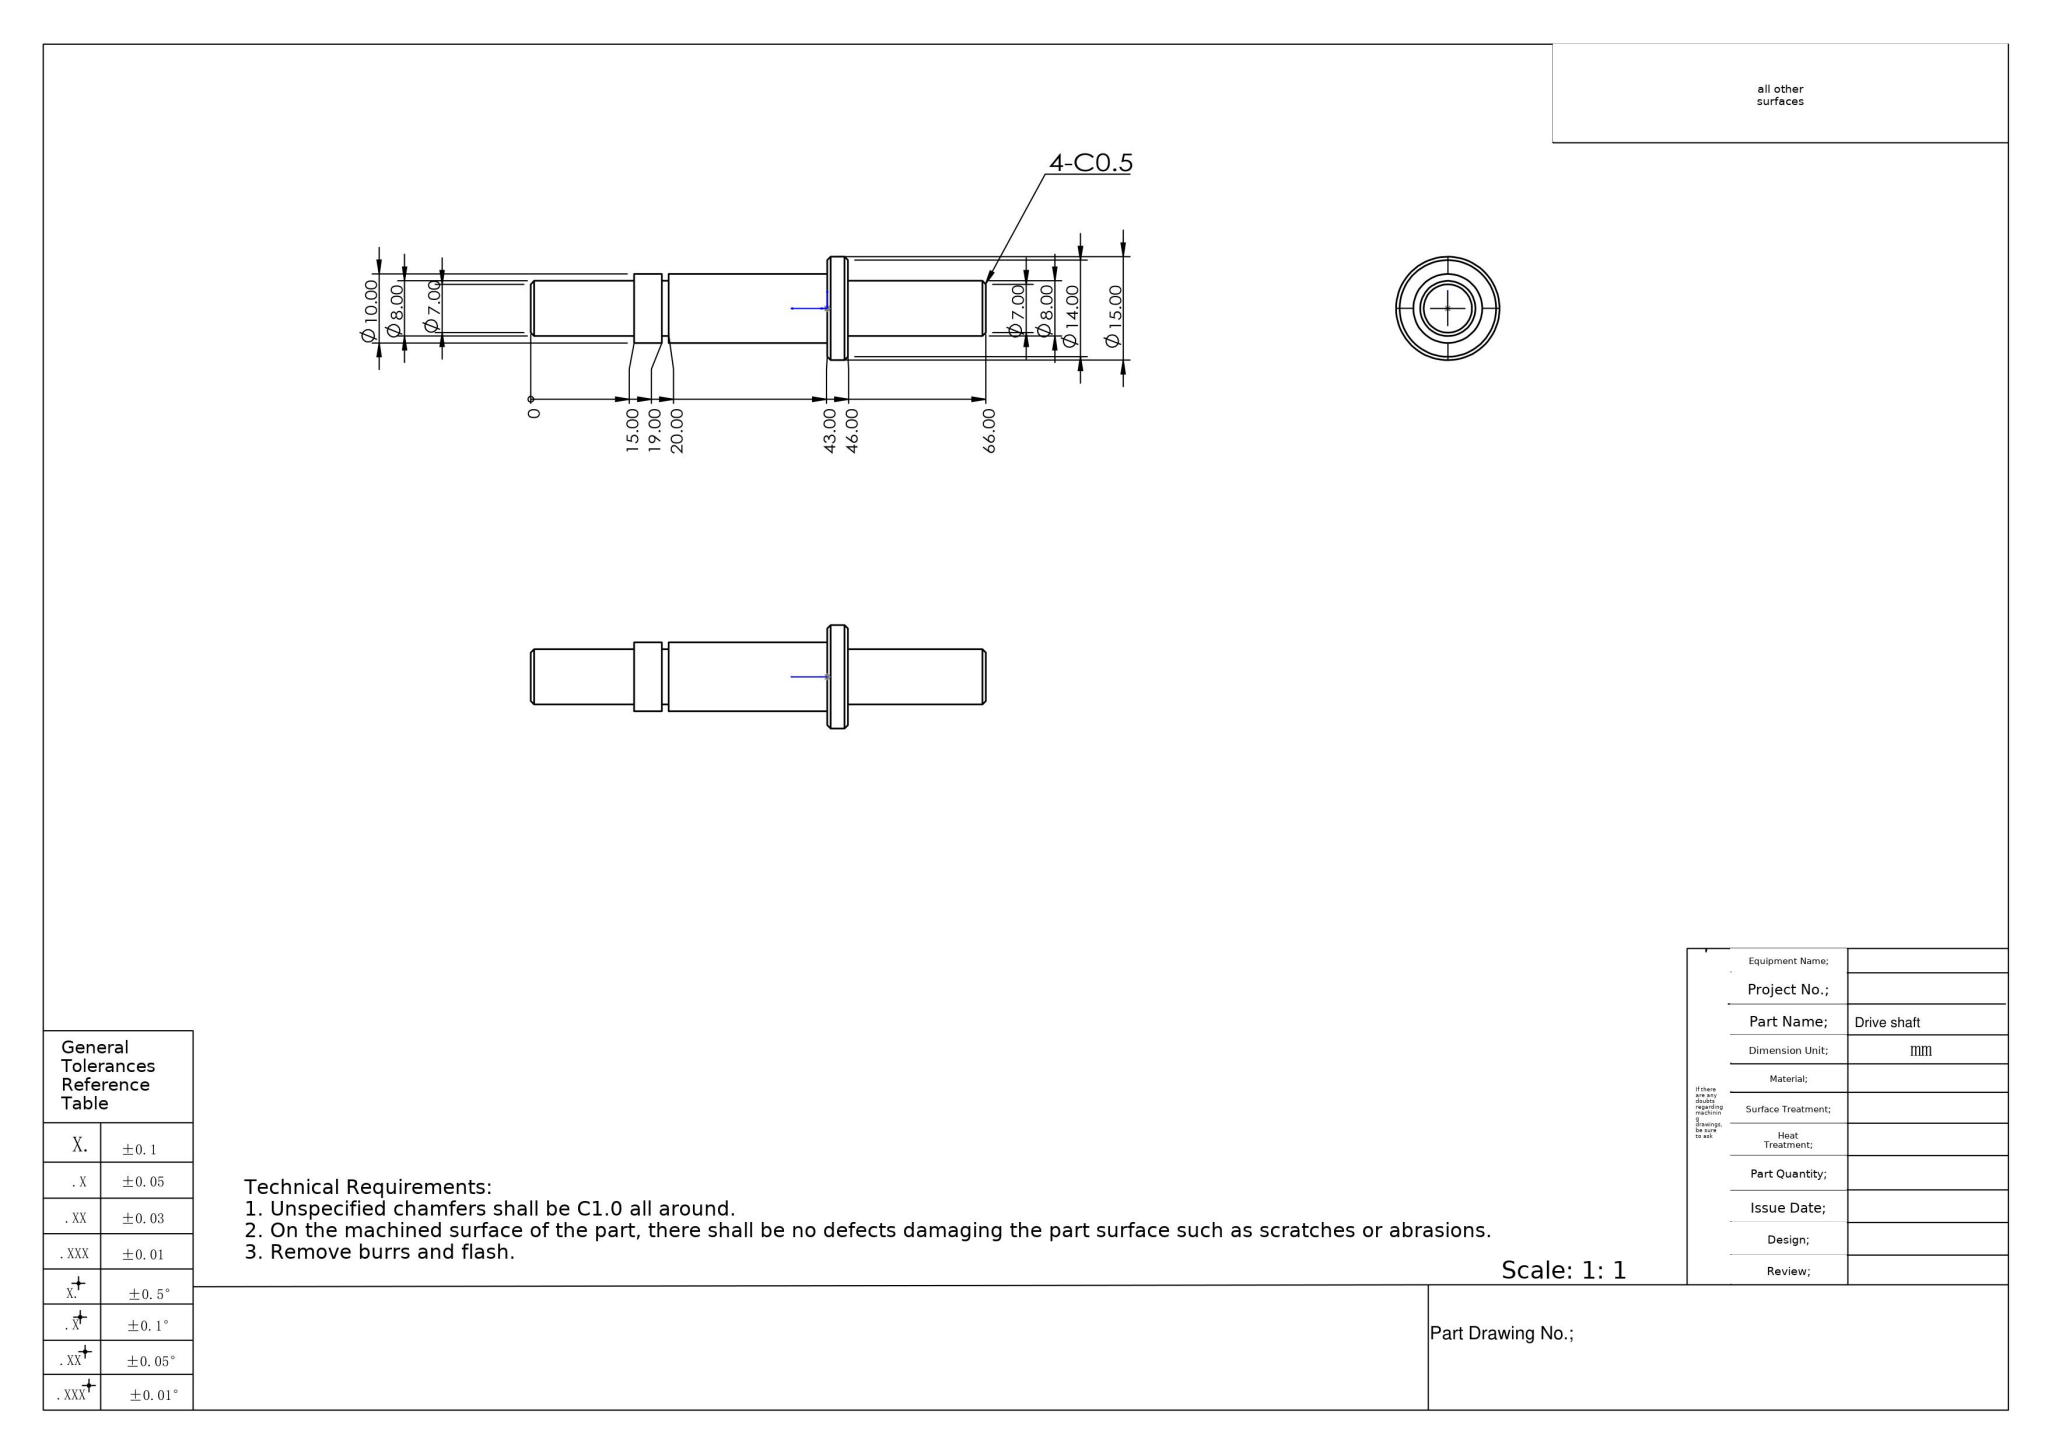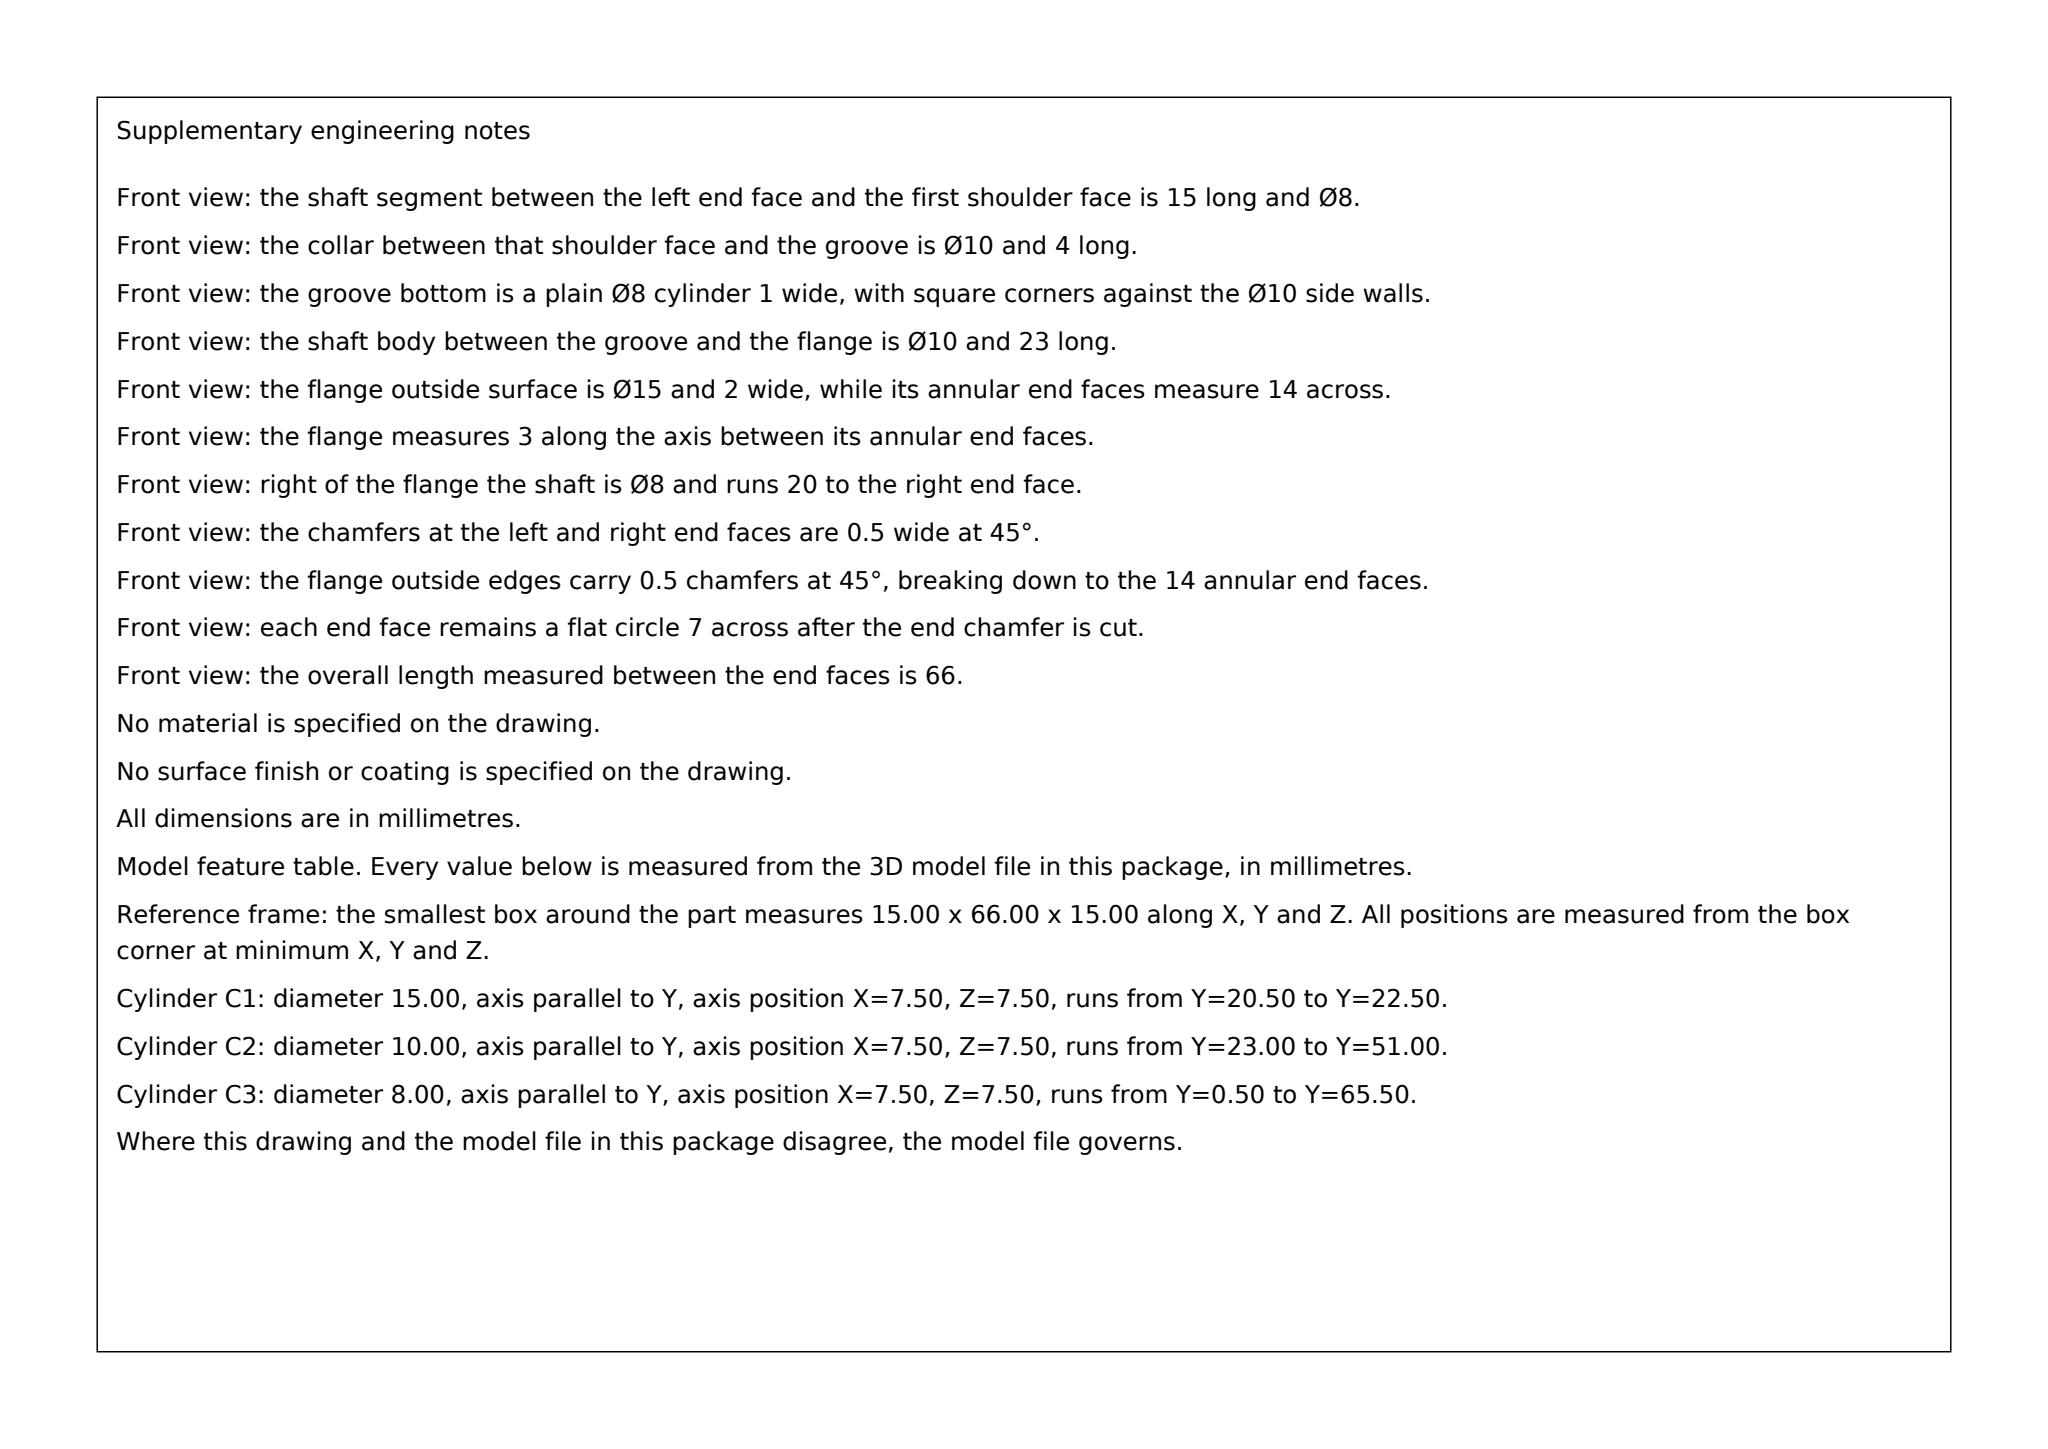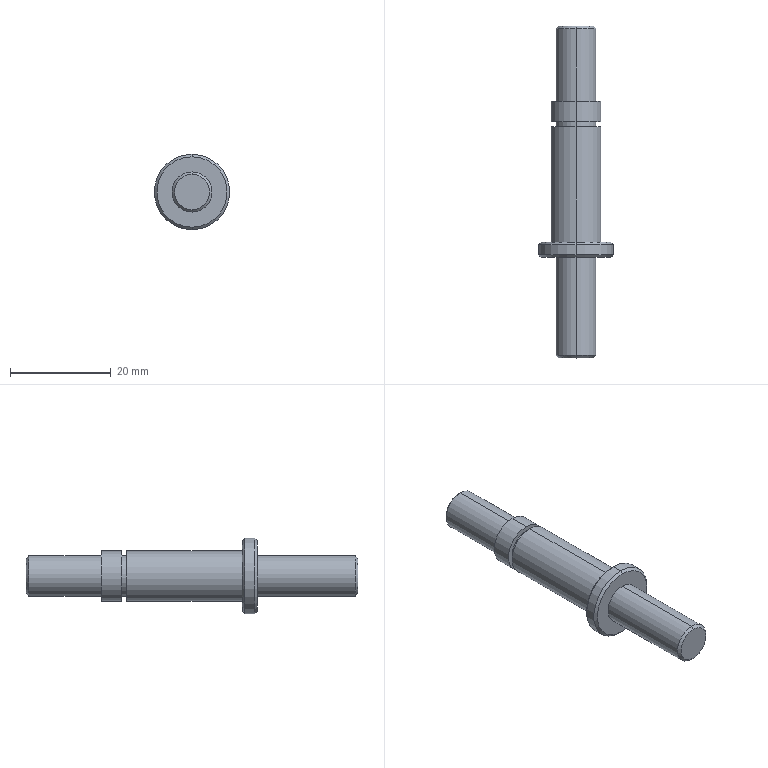Part | SolidWorks | mm | 1 solid | 27 faces | box 15 x 66 x 15 mm | volume 4443 mm3 | cylinder 12 | cone 8 | plane 7 | commonest cylinder face diameters 8 x6 10 x4 15 x2
build123d program:
from build123d import *

# Parameters (mm, degrees)
SKETCH1_R           = 5
BOSS_EXTRUDE1_DEPTH = 28
SKETCH2_R           = 7.5
BOSS_EXTRUDE2_DEPTH = 3
CHAMFER1_SIZE       = 0.5
SKETCH3_R           = 4
BOSS_EXTRUDE3_DEPTH = 20
CHAMFER2_SIZE       = 0.5
BOSS_EXTRUDE4_START = 15
SKETCH4_R           = 4
BOSS_EXTRUDE4_DEPTH = 15
CHAMFER3_SIZE       = 0.5
SKETCH5_W           = 1
SKETCH5_H           = 1


with BuildPart() as part:
    # Sketch1 → Boss-Extrude1 (new body)
    with BuildSketch(Plane(origin=(0, 0, 0), x_dir=(1, 0, 0), z_dir=(0, 1, 0))):
        with Locations(Location((0, 0, 0), (0, 0, 270))):
            Circle(SKETCH1_R)
    extrude(amount=BOSS_EXTRUDE1_DEPTH)

    # Sketch2 → Boss-Extrude2 (add)
    with BuildSketch(Plane.XZ):
        with Locations(Location((0, 0, 0), (0, 0, 270))):
            Circle(SKETCH2_R)
    extrude(amount=BOSS_EXTRUDE2_DEPTH)

    # Chamfer1
    chamfer1_edges = [part.edges().sort_by_distance(p)[0] for p in [
        (0, 0, 7.5),
        (0, -3, 7.5),
    ]]
    chamfer(chamfer1_edges, length=CHAMFER1_SIZE)

    # Sketch3 → Boss-Extrude3 (add)
    with BuildSketch(Plane.XZ.offset(3)):
        with Locations(Location((0, 0, 0), (0, 0, 270))):
            Circle(SKETCH3_R)
    extrude(amount=BOSS_EXTRUDE3_DEPTH)

    # Chamfer2
    chamfer2_edges = [part.edges().sort_by_distance(p)[0] for p in [
        (0, -23, 4),
    ]]
    chamfer(chamfer2_edges, length=CHAMFER2_SIZE)

    # Sketch4 → Boss-Extrude4 (add)
    with BuildSketch(Plane(origin=(0, 28, 0), x_dir=(1, 0, 0), z_dir=(0, 1, 0)).offset(BOSS_EXTRUDE4_START)):
        with Locations(Location((0, 0, 0), (0, 0, 90))):
            Circle(SKETCH4_R)
    extrude(amount=-BOSS_EXTRUDE4_DEPTH)

    # Chamfer3
    chamfer3_edges = [part.edges().sort_by_distance(p)[0] for p in [
        (0, 43, 4),
    ]]
    chamfer(chamfer3_edges, length=CHAMFER3_SIZE)

    # Sketch5 → Cut-Revolve1 (revolve, cut)
    with BuildSketch(Plane(origin=(0, 0, 0), x_dir=(0, 0, -1), z_dir=(1, 0, 0)), mode=Mode.PRIVATE) as cut_revolve1_sk:
        with Locations((-4.5, 23.5)):
            Rectangle(SKETCH5_W, SKETCH5_H)
    revolve(cut_revolve1_sk.sketch.rotate(Axis((0, 0, 0), (0, 1, 0)), 180), axis=Axis((0, 0, 0), (0, 1, 0)), mode=Mode.SUBTRACT)


solid = part.part
STEP:
#1=CARTESIAN_POINT('',(0.,28.,5.));
#2=VERTEX_POINT('',#1);
#3=CARTESIAN_POINT('',(0.,28.,-5.));
#4=VERTEX_POINT('',#3);
#5=CARTESIAN_POINT('',(0.,28.,0.));
#6=DIRECTION('',(0.,1.,0.));
#7=DIRECTION('',(0.,0.,1.));
#8=AXIS2_PLACEMENT_3D('',#5,#6,#7);
#9=CIRCLE('',#8,5.);
#10=EDGE_CURVE('',#2,#4,#9,.T.);
#11=ORIENTED_EDGE('',*,*,#10,.F.);
#12=CARTESIAN_POINT('',(0.,24.,5.));
#13=VERTEX_POINT('',#12);
#14=CARTESIAN_POINT('',(0.,28.,5.));
#15=DIRECTION('',(0.,-1.,0.));
#16=VECTOR('',#15,1000.);
#17=LINE('',#14,#16);
#18=EDGE_CURVE('',#2,#13,#17,.T.);
#19=ORIENTED_EDGE('',*,*,#18,.T.);
#20=CARTESIAN_POINT('',(0.,24.,-5.));
#21=VERTEX_POINT('',#20);
#22=CARTESIAN_POINT('',(0.,24.,0.));
#23=DIRECTION('',(0.,-1.,0.));
#24=DIRECTION('',(0.,0.,-1.));
#25=AXIS2_PLACEMENT_3D('',#22,#23,#24);
#26=CIRCLE('',#25,5.);
#27=EDGE_CURVE('',#21,#13,#26,.T.);
#28=ORIENTED_EDGE('',*,*,#27,.F.);
#29=CARTESIAN_POINT('',(0.,28.,-5.));
#30=DIRECTION('',(0.,-1.,0.));
#31=VECTOR('',#30,1000.);
#32=LINE('',#29,#31);
#33=EDGE_CURVE('',#4,#21,#32,.T.);
#34=ORIENTED_EDGE('',*,*,#33,.F.);
#35=EDGE_LOOP('',(#11,#19,#28,#34));
#36=FACE_OUTER_BOUND('',#35,.T.);
#37=CARTESIAN_POINT('',(0.,28.,0.));
#38=DIRECTION('',(0.,-1.,0.));
#39=DIRECTION('',(0.,0.,-1.));
#40=AXIS2_PLACEMENT_3D('',#37,#38,#39);
#41=CYLINDRICAL_SURFACE('',#40,5.);
#42=ADVANCED_FACE('',(#36),#41,.T.);
#43=CARTESIAN_POINT('',(0.,42.5,-4.));
#44=VERTEX_POINT('',#43);
#45=CARTESIAN_POINT('',(0.,42.5,4.));
#46=VERTEX_POINT('',#45);
#47=CARTESIAN_POINT('',(0.,42.5,0.));
#48=DIRECTION('',(0.,-1.,0.));
#49=DIRECTION('',(0.,0.,1.));
#50=AXIS2_PLACEMENT_3D('',#47,#48,#49);
#51=CIRCLE('',#50,4.);
#52=EDGE_CURVE('',#44,#46,#51,.T.);
#53=ORIENTED_EDGE('',*,*,#52,.T.);
#54=CARTESIAN_POINT('',(0.,28.,4.));
#55=VERTEX_POINT('',#54);
#56=CARTESIAN_POINT('',(0.,43.,4.));
#57=DIRECTION('',(0.,-1.,0.));
#58=VECTOR('',#57,1000.);
#59=LINE('',#56,#58);
#60=EDGE_CURVE('',#46,#55,#59,.T.);
#61=ORIENTED_EDGE('',*,*,#60,.T.);
#62=CARTESIAN_POINT('',(0.,28.,-4.));
#63=VERTEX_POINT('',#62);
#64=CARTESIAN_POINT('',(0.,28.,0.));
#65=DIRECTION('',(0.,1.,0.));
#66=DIRECTION('',(0.,0.,1.));
#67=AXIS2_PLACEMENT_3D('',#64,#65,#66);
#68=CIRCLE('',#67,4.);
#69=EDGE_CURVE('',#55,#63,#68,.T.);
#70=ORIENTED_EDGE('',*,*,#69,.T.);
#71=CARTESIAN_POINT('',(0.,43.,-4.));
#72=DIRECTION('',(0.,-1.,0.));
#73=VECTOR('',#72,1000.);
#74=LINE('',#71,#73);
#75=EDGE_CURVE('',#44,#63,#74,.T.);
#76=ORIENTED_EDGE('',*,*,#75,.F.);
#77=EDGE_LOOP('',(#53,#61,#70,#76));
#78=FACE_OUTER_BOUND('',#77,.T.);
#79=CARTESIAN_POINT('',(0.,43.,0.));
#80=DIRECTION('',(0.,-1.,0.));
#81=DIRECTION('',(0.,0.,-1.));
#82=AXIS2_PLACEMENT_3D('',#79,#80,#81);
#83=CYLINDRICAL_SURFACE('',#82,4.);
#84=ADVANCED_FACE('',(#78),#83,.T.);
#85=CARTESIAN_POINT('',(0.,43.,3.5));
#86=VERTEX_POINT('',#85);
#87=CARTESIAN_POINT('',(0.,43.,-3.5));
#88=VERTEX_POINT('',#87);
#89=CARTESIAN_POINT('',(0.,43.,0.));
#90=DIRECTION('',(0.,1.,0.));
#91=DIRECTION('',(0.,0.,1.));
#92=AXIS2_PLACEMENT_3D('',#89,#90,#91);
#93=CIRCLE('',#92,3.5);
#94=EDGE_CURVE('',#86,#88,#93,.T.);
#95=ORIENTED_EDGE('',*,*,#94,.F.);
#96=CARTESIAN_POINT('',(0.,43.,3.5));
#97=DIRECTION('',(0.,-0.7071,0.7071));
#98=VECTOR('',#97,1000.);
#99=LINE('',#96,#98);
#100=EDGE_CURVE('',#86,#46,#99,.T.);
#101=ORIENTED_EDGE('',*,*,#100,.T.);
#102=ORIENTED_EDGE('',*,*,#52,.F.);
#103=CARTESIAN_POINT('',(0.,43.,-3.5));
#104=DIRECTION('',(0.,-0.7071,-0.7071));
#105=VECTOR('',#104,1000.);
#106=LINE('',#103,#105);
#107=EDGE_CURVE('',#88,#44,#106,.T.);
#108=ORIENTED_EDGE('',*,*,#107,.F.);
#109=EDGE_LOOP('',(#95,#101,#102,#108));
#110=FACE_OUTER_BOUND('',#109,.T.);
#111=CARTESIAN_POINT('',(0.,43.,0.));
#112=DIRECTION('',(0.,-1.,0.));
#113=DIRECTION('',(0.,0.,-1.));
#114=AXIS2_PLACEMENT_3D('',#111,#112,#113);
#115=CONICAL_SURFACE('',#114,3.5,0.7854);
#116=ADVANCED_FACE('',(#110),#115,.T.);
#117=CARTESIAN_POINT('',(0.,24.,-4.));
#118=VERTEX_POINT('',#117);
#119=CARTESIAN_POINT('',(0.,24.,4.));
#120=VERTEX_POINT('',#119);
#121=CARTESIAN_POINT('',(0.,24.,0.));
#122=DIRECTION('',(0.,-1.,0.));
#123=DIRECTION('',(0.,0.,-1.));
#124=AXIS2_PLACEMENT_3D('',#121,#122,#123);
#125=CIRCLE('',#124,4.);
#126=EDGE_CURVE('',#118,#120,#125,.T.);
#127=ORIENTED_EDGE('',*,*,#126,.T.);
#128=CARTESIAN_POINT('',(0.,23.,4.));
#129=VERTEX_POINT('',#128);
#130=CARTESIAN_POINT('',(0.,0.,4.));
#131=DIRECTION('',(0.,-1.,0.));
#132=VECTOR('',#131,1000.);
#133=LINE('',#130,#132);
#134=EDGE_CURVE('',#120,#129,#133,.T.);
#135=ORIENTED_EDGE('',*,*,#134,.T.);
#136=CARTESIAN_POINT('',(0.,23.,-4.));
#137=VERTEX_POINT('',#136);
#138=CARTESIAN_POINT('',(0.,23.,0.));
#139=DIRECTION('',(0.,-1.,0.));
#140=DIRECTION('',(0.,0.,-1.));
#141=AXIS2_PLACEMENT_3D('',#138,#139,#140);
#142=CIRCLE('',#141,4.);
#143=EDGE_CURVE('',#137,#129,#142,.T.);
#144=ORIENTED_EDGE('',*,*,#143,.F.);
#145=CARTESIAN_POINT('',(0.,0.,-4.));
#146=DIRECTION('',(0.,-1.,0.));
#147=VECTOR('',#146,1000.);
#148=LINE('',#145,#147);
#149=EDGE_CURVE('',#118,#137,#148,.T.);
#150=ORIENTED_EDGE('',*,*,#149,.F.);
#151=EDGE_LOOP('',(#127,#135,#144,#150));
#152=FACE_OUTER_BOUND('',#151,.T.);
#153=CARTESIAN_POINT('',(0.,0.,0.));
#154=DIRECTION('',(0.,-1.,0.));
#155=DIRECTION('',(0.,0.,-1.));
#156=AXIS2_PLACEMENT_3D('',#153,#154,#155);
#157=CYLINDRICAL_SURFACE('',#156,4.);
#158=ADVANCED_FACE('',(#152),#157,.T.);
#159=CARTESIAN_POINT('',(0.,-23.,-3.5));
#160=VERTEX_POINT('',#159);
#161=CARTESIAN_POINT('',(0.,-23.,3.5));
#162=VERTEX_POINT('',#161);
#163=CARTESIAN_POINT('',(0.,-23.,0.));
#164=DIRECTION('',(0.,-1.,0.));
#165=DIRECTION('',(0.,0.,-1.));
#166=AXIS2_PLACEMENT_3D('',#163,#164,#165);
#167=CIRCLE('',#166,3.5);
#168=EDGE_CURVE('',#160,#162,#167,.T.);
#169=ORIENTED_EDGE('',*,*,#168,.F.);
#170=CARTESIAN_POINT('',(0.,-22.5,-4.));
#171=VERTEX_POINT('',#170);
#172=CARTESIAN_POINT('',(0.,-23.,-3.5));
#173=DIRECTION('',(0.,0.7071,-0.7071));
#174=VECTOR('',#173,1000.);
#175=LINE('',#172,#174);
#176=EDGE_CURVE('',#160,#171,#175,.T.);
#177=ORIENTED_EDGE('',*,*,#176,.T.);
#178=CARTESIAN_POINT('',(0.,-22.5,4.));
#179=VERTEX_POINT('',#178);
#180=CARTESIAN_POINT('',(0.,-22.5,0.));
#181=DIRECTION('',(0.,1.,0.));
#182=DIRECTION('',(0.,0.,-1.));
#183=AXIS2_PLACEMENT_3D('',#180,#181,#182);
#184=CIRCLE('',#183,4.);
#185=EDGE_CURVE('',#179,#171,#184,.T.);
#186=ORIENTED_EDGE('',*,*,#185,.F.);
#187=CARTESIAN_POINT('',(0.,-23.,3.5));
#188=DIRECTION('',(0.,0.7071,0.7071));
#189=VECTOR('',#188,1000.);
#190=LINE('',#187,#189);
#191=EDGE_CURVE('',#162,#179,#190,.T.);
#192=ORIENTED_EDGE('',*,*,#191,.F.);
#193=EDGE_LOOP('',(#169,#177,#186,#192));
#194=FACE_OUTER_BOUND('',#193,.T.);
#195=CARTESIAN_POINT('',(0.,-23.,0.));
#196=DIRECTION('',(0.,1.,0.));
#197=DIRECTION('',(0.,0.,1.));
#198=AXIS2_PLACEMENT_3D('',#195,#196,#197);
#199=CONICAL_SURFACE('',#198,3.5,0.7854);
#200=ADVANCED_FACE('',(#194),#199,.T.);
#201=ORIENTED_EDGE('',*,*,#185,.T.);
#202=CARTESIAN_POINT('',(0.,-3.,-4.));
#203=VERTEX_POINT('',#202);
#204=CARTESIAN_POINT('',(0.,-23.,-4.));
#205=DIRECTION('',(0.,1.,0.));
#206=VECTOR('',#205,1000.);
#207=LINE('',#204,#206);
#208=EDGE_CURVE('',#171,#203,#207,.T.);
#209=ORIENTED_EDGE('',*,*,#208,.T.);
#210=CARTESIAN_POINT('',(0.,-3.,4.));
#211=VERTEX_POINT('',#210);
#212=CARTESIAN_POINT('',(0.,-3.,0.));
#213=DIRECTION('',(0.,-1.,0.));
#214=DIRECTION('',(0.,0.,-1.));
#215=AXIS2_PLACEMENT_3D('',#212,#213,#214);
#216=CIRCLE('',#215,4.);
#217=EDGE_CURVE('',#203,#211,#216,.T.);
#218=ORIENTED_EDGE('',*,*,#217,.T.);
#219=CARTESIAN_POINT('',(0.,-23.,4.));
#220=DIRECTION('',(0.,1.,0.));
#221=VECTOR('',#220,1000.);
#222=LINE('',#219,#221);
#223=EDGE_CURVE('',#179,#211,#222,.T.);
#224=ORIENTED_EDGE('',*,*,#223,.F.);
#225=EDGE_LOOP('',(#201,#209,#218,#224));
#226=FACE_OUTER_BOUND('',#225,.T.);
#227=CARTESIAN_POINT('',(0.,-23.,0.));
#228=DIRECTION('',(0.,1.,0.));
#229=DIRECTION('',(0.,0.,1.));
#230=AXIS2_PLACEMENT_3D('',#227,#228,#229);
#231=CYLINDRICAL_SURFACE('',#230,4.);
#232=ADVANCED_FACE('',(#226),#231,.T.);
#233=CARTESIAN_POINT('',(0.,-3.,-7.));
#234=VERTEX_POINT('',#233);
#235=CARTESIAN_POINT('',(0.,-3.,7.));
#236=VERTEX_POINT('',#235);
#237=CARTESIAN_POINT('',(0.,-3.,0.));
#238=DIRECTION('',(0.,-1.,0.));
#239=DIRECTION('',(0.,0.,-1.));
#240=AXIS2_PLACEMENT_3D('',#237,#238,#239);
#241=CIRCLE('',#240,7.);
#242=EDGE_CURVE('',#234,#236,#241,.T.);
#243=ORIENTED_EDGE('',*,*,#242,.F.);
#244=CARTESIAN_POINT('',(0.,-2.5,-7.5));
#245=VERTEX_POINT('',#244);
#246=CARTESIAN_POINT('',(0.,-3.,-7.));
#247=DIRECTION('',(0.,0.7071,-0.7071));
#248=VECTOR('',#247,1000.);
#249=LINE('',#246,#248);
#250=EDGE_CURVE('',#234,#245,#249,.T.);
#251=ORIENTED_EDGE('',*,*,#250,.T.);
#252=CARTESIAN_POINT('',(0.,-2.5,7.5));
#253=VERTEX_POINT('',#252);
#254=CARTESIAN_POINT('',(0.,-2.5,0.));
#255=DIRECTION('',(0.,1.,0.));
#256=DIRECTION('',(0.,0.,-1.));
#257=AXIS2_PLACEMENT_3D('',#254,#255,#256);
#258=CIRCLE('',#257,7.5);
#259=EDGE_CURVE('',#253,#245,#258,.T.);
#260=ORIENTED_EDGE('',*,*,#259,.F.);
#261=CARTESIAN_POINT('',(0.,-3.,7.));
#262=DIRECTION('',(0.,0.7071,0.7071));
#263=VECTOR('',#262,1000.);
#264=LINE('',#261,#263);
#265=EDGE_CURVE('',#236,#253,#264,.T.);
#266=ORIENTED_EDGE('',*,*,#265,.F.);
#267=EDGE_LOOP('',(#243,#251,#260,#266));
#268=FACE_OUTER_BOUND('',#267,.T.);
#269=CARTESIAN_POINT('',(0.,-3.,0.));
#270=DIRECTION('',(0.,1.,0.));
#271=DIRECTION('',(0.,0.,1.));
#272=AXIS2_PLACEMENT_3D('',#269,#270,#271);
#273=CONICAL_SURFACE('',#272,7.,0.7854);
#274=ADVANCED_FACE('',(#268),#273,.T.);
#275=CARTESIAN_POINT('',(0.,0.,7.));
#276=VERTEX_POINT('',#275);
#277=CARTESIAN_POINT('',(0.,0.,-7.));
#278=VERTEX_POINT('',#277);
#279=CARTESIAN_POINT('',(0.,0.,0.));
#280=DIRECTION('',(0.,1.,0.));
#281=DIRECTION('',(0.,0.,-1.));
#282=AXIS2_PLACEMENT_3D('',#279,#280,#281);
#283=CIRCLE('',#282,7.);
#284=EDGE_CURVE('',#276,#278,#283,.T.);
#285=ORIENTED_EDGE('',*,*,#284,.F.);
#286=CARTESIAN_POINT('',(0.,-0.5,7.5));
#287=VERTEX_POINT('',#286);
#288=CARTESIAN_POINT('',(0.,-0.5,7.5));
#289=DIRECTION('',(0.,-0.7071,0.7071));
#290=VECTOR('',#289,1000.);
#291=LINE('',#288,#290);
#292=EDGE_CURVE('',#276,#287,#291,.T.);
#293=ORIENTED_EDGE('',*,*,#292,.T.);
#294=CARTESIAN_POINT('',(0.,-0.5,-7.5));
#295=VERTEX_POINT('',#294);
#296=CARTESIAN_POINT('',(0.,-0.5,0.));
#297=DIRECTION('',(0.,-1.,0.));
#298=DIRECTION('',(0.,0.,-1.));
#299=AXIS2_PLACEMENT_3D('',#296,#297,#298);
#300=CIRCLE('',#299,7.5);
#301=EDGE_CURVE('',#295,#287,#300,.T.);
#302=ORIENTED_EDGE('',*,*,#301,.F.);
#303=CARTESIAN_POINT('',(0.,-0.5,-7.5));
#304=DIRECTION('',(0.,-0.7071,-0.7071));
#305=VECTOR('',#304,1000.);
#306=LINE('',#303,#305);
#307=EDGE_CURVE('',#278,#295,#306,.T.);
#308=ORIENTED_EDGE('',*,*,#307,.F.);
#309=EDGE_LOOP('',(#285,#293,#302,#308));
#310=FACE_OUTER_BOUND('',#309,.T.);
#311=CARTESIAN_POINT('',(0.,-0.5,0.));
#312=DIRECTION('',(0.,-1.,0.));
#313=DIRECTION('',(0.,0.,-1.));
#314=AXIS2_PLACEMENT_3D('',#311,#312,#313);
#315=CONICAL_SURFACE('',#314,7.5,0.7854);
#316=ADVANCED_FACE('',(#310),#315,.T.);
#317=ORIENTED_EDGE('',*,*,#259,.T.);
#318=CARTESIAN_POINT('',(0.,-3.,-7.5));
#319=DIRECTION('',(0.,1.,0.));
#320=VECTOR('',#319,1000.);
#321=LINE('',#318,#320);
#322=EDGE_CURVE('',#245,#295,#321,.T.);
#323=ORIENTED_EDGE('',*,*,#322,.T.);
#324=ORIENTED_EDGE('',*,*,#301,.T.);
#325=CARTESIAN_POINT('',(0.,-3.,7.5));
#326=DIRECTION('',(0.,1.,0.));
#327=VECTOR('',#326,1000.);
#328=LINE('',#325,#327);
#329=EDGE_CURVE('',#253,#287,#328,.T.);
#330=ORIENTED_EDGE('',*,*,#329,.F.);
#331=EDGE_LOOP('',(#317,#323,#324,#330));
#332=FACE_OUTER_BOUND('',#331,.T.);
#333=CARTESIAN_POINT('',(0.,-3.,0.));
#334=DIRECTION('',(0.,1.,0.));
#335=DIRECTION('',(0.,0.,1.));
#336=AXIS2_PLACEMENT_3D('',#333,#334,#335);
#337=CYLINDRICAL_SURFACE('',#336,7.5);
#338=ADVANCED_FACE('',(#332),#337,.T.);
#339=CARTESIAN_POINT('',(0.,23.,-5.));
#340=VERTEX_POINT('',#339);
#341=CARTESIAN_POINT('',(0.,23.,5.));
#342=VERTEX_POINT('',#341);
#343=CARTESIAN_POINT('',(0.,23.,0.));
#344=DIRECTION('',(0.,-1.,0.));
#345=DIRECTION('',(0.,0.,-1.));
#346=AXIS2_PLACEMENT_3D('',#343,#344,#345);
#347=CIRCLE('',#346,5.);
#348=EDGE_CURVE('',#340,#342,#347,.T.);
#349=ORIENTED_EDGE('',*,*,#348,.T.);
#350=CARTESIAN_POINT('',(0.,0.,5.));
#351=VERTEX_POINT('',#350);
#352=CARTESIAN_POINT('',(0.,28.,5.));
#353=DIRECTION('',(0.,-1.,0.));
#354=VECTOR('',#353,1000.);
#355=LINE('',#352,#354);
#356=EDGE_CURVE('',#342,#351,#355,.T.);
#357=ORIENTED_EDGE('',*,*,#356,.T.);
#358=CARTESIAN_POINT('',(0.,0.,-5.));
#359=VERTEX_POINT('',#358);
#360=CARTESIAN_POINT('',(0.,0.,0.));
#361=DIRECTION('',(0.,-1.,0.));
#362=DIRECTION('',(0.,0.,-1.));
#363=AXIS2_PLACEMENT_3D('',#360,#361,#362);
#364=CIRCLE('',#363,5.);
#365=EDGE_CURVE('',#359,#351,#364,.T.);
#366=ORIENTED_EDGE('',*,*,#365,.F.);
#367=CARTESIAN_POINT('',(0.,28.,-5.));
#368=DIRECTION('',(0.,-1.,0.));
#369=VECTOR('',#368,1000.);
#370=LINE('',#367,#369);
#371=EDGE_CURVE('',#340,#359,#370,.T.);
#372=ORIENTED_EDGE('',*,*,#371,.F.);
#373=EDGE_LOOP('',(#349,#357,#366,#372));
#374=FACE_OUTER_BOUND('',#373,.T.);
#375=CARTESIAN_POINT('',(0.,28.,0.));
#376=DIRECTION('',(0.,-1.,0.));
#377=DIRECTION('',(0.,0.,-1.));
#378=AXIS2_PLACEMENT_3D('',#375,#376,#377);
#379=CYLINDRICAL_SURFACE('',#378,5.);
#380=ADVANCED_FACE('',(#374),#379,.T.);
#381=ORIENTED_EDGE('',*,*,#356,.F.);
#382=CARTESIAN_POINT('',(0.,23.,0.));
#383=DIRECTION('',(0.,-1.,0.));
#384=DIRECTION('',(0.,0.,-1.));
#385=AXIS2_PLACEMENT_3D('',#382,#383,#384);
#386=CIRCLE('',#385,5.);
#387=EDGE_CURVE('',#342,#340,#386,.T.);
#388=ORIENTED_EDGE('',*,*,#387,.T.);
#389=ORIENTED_EDGE('',*,*,#371,.T.);
#390=CARTESIAN_POINT('',(0.,0.,0.));
#391=DIRECTION('',(0.,-1.,0.));
#392=DIRECTION('',(0.,0.,-1.));
#393=AXIS2_PLACEMENT_3D('',#390,#391,#392);
#394=CIRCLE('',#393,5.);
#395=EDGE_CURVE('',#351,#359,#394,.T.);
#396=ORIENTED_EDGE('',*,*,#395,.F.);
#397=EDGE_LOOP('',(#381,#388,#389,#396));
#398=FACE_OUTER_BOUND('',#397,.T.);
#399=CARTESIAN_POINT('',(0.,28.,0.));
#400=DIRECTION('',(0.,-1.,0.));
#401=DIRECTION('',(0.,0.,-1.));
#402=AXIS2_PLACEMENT_3D('',#399,#400,#401);
#403=CYLINDRICAL_SURFACE('',#402,5.);
#404=ADVANCED_FACE('',(#398),#403,.T.);
#405=CARTESIAN_POINT('',(0.,-3.,0.));
#406=DIRECTION('',(0.,-1.,0.));
#407=DIRECTION('',(0.,0.,-1.));
#408=AXIS2_PLACEMENT_3D('',#405,#406,#407);
#409=CIRCLE('',#408,7.);
#410=EDGE_CURVE('',#236,#234,#409,.T.);
#411=ORIENTED_EDGE('',*,*,#410,.T.);
#412=ORIENTED_EDGE('',*,*,#242,.T.);
#413=EDGE_LOOP('',(#411,#412));
#414=FACE_OUTER_BOUND('',#413,.T.);
#415=CARTESIAN_POINT('',(0.,-3.,0.));
#416=DIRECTION('',(0.,-1.,0.));
#417=DIRECTION('',(0.,0.,-1.));
#418=AXIS2_PLACEMENT_3D('',#415,#416,#417);
#419=CIRCLE('',#418,4.);
#420=EDGE_CURVE('',#211,#203,#419,.T.);
#421=ORIENTED_EDGE('',*,*,#420,.F.);
#422=ORIENTED_EDGE('',*,*,#217,.F.);
#423=EDGE_LOOP('',(#421,#422));
#424=FACE_BOUND('',#423,.T.);
#425=CARTESIAN_POINT('',(0.,-3.,0.));
#426=DIRECTION('',(0.,-1.,0.));
#427=DIRECTION('',(0.,0.,-1.));
#428=AXIS2_PLACEMENT_3D('',#425,#426,#427);
#429=PLANE('',#428);
#430=ADVANCED_FACE('',(#414,#424),#429,.T.);
#431=CARTESIAN_POINT('',(0.,0.,0.));
#432=DIRECTION('',(0.,1.,0.));
#433=DIRECTION('',(0.,0.,-1.));
#434=AXIS2_PLACEMENT_3D('',#431,#432,#433);
#435=CIRCLE('',#434,7.);
#436=EDGE_CURVE('',#278,#276,#435,.T.);
#437=ORIENTED_EDGE('',*,*,#436,.T.);
#438=ORIENTED_EDGE('',*,*,#284,.T.);
#439=EDGE_LOOP('',(#437,#438));
#440=FACE_OUTER_BOUND('',#439,.T.);
#441=ORIENTED_EDGE('',*,*,#365,.T.);
#442=ORIENTED_EDGE('',*,*,#395,.T.);
#443=EDGE_LOOP('',(#441,#442));
#444=FACE_BOUND('',#443,.T.);
#445=CARTESIAN_POINT('',(0.,0.,0.));
#446=DIRECTION('',(0.,-1.,0.));
#447=DIRECTION('',(0.,0.,-1.));
#448=AXIS2_PLACEMENT_3D('',#445,#446,#447);
#449=PLANE('',#448);
#450=ADVANCED_FACE('',(#440,#444),#449,.F.);
#451=ORIENTED_EDGE('',*,*,#322,.F.);
#452=CARTESIAN_POINT('',(0.,-2.5,0.));
#453=DIRECTION('',(0.,1.,0.));
#454=DIRECTION('',(0.,0.,-1.));
#455=AXIS2_PLACEMENT_3D('',#452,#453,#454);
#456=CIRCLE('',#455,7.5);
#457=EDGE_CURVE('',#245,#253,#456,.T.);
#458=ORIENTED_EDGE('',*,*,#457,.T.);
#459=ORIENTED_EDGE('',*,*,#329,.T.);
#460=CARTESIAN_POINT('',(0.,-0.5,0.));
#461=DIRECTION('',(0.,-1.,0.));
#462=DIRECTION('',(0.,0.,-1.));
#463=AXIS2_PLACEMENT_3D('',#460,#461,#462);
#464=CIRCLE('',#463,7.5);
#465=EDGE_CURVE('',#287,#295,#464,.T.);
#466=ORIENTED_EDGE('',*,*,#465,.T.);
#467=EDGE_LOOP('',(#451,#458,#459,#466));
#468=FACE_OUTER_BOUND('',#467,.T.);
#469=CARTESIAN_POINT('',(0.,-3.,0.));
#470=DIRECTION('',(0.,1.,0.));
#471=DIRECTION('',(0.,0.,1.));
#472=AXIS2_PLACEMENT_3D('',#469,#470,#471);
#473=CYLINDRICAL_SURFACE('',#472,7.5);
#474=ADVANCED_FACE('',(#468),#473,.T.);
#475=ORIENTED_EDGE('',*,*,#292,.F.);
#476=ORIENTED_EDGE('',*,*,#436,.F.);
#477=ORIENTED_EDGE('',*,*,#307,.T.);
#478=ORIENTED_EDGE('',*,*,#465,.F.);
#479=EDGE_LOOP('',(#475,#476,#477,#478));
#480=FACE_OUTER_BOUND('',#479,.T.);
#481=CARTESIAN_POINT('',(0.,-0.5,0.));
#482=DIRECTION('',(0.,-1.,0.));
#483=DIRECTION('',(0.,0.,-1.));
#484=AXIS2_PLACEMENT_3D('',#481,#482,#483);
#485=CONICAL_SURFACE('',#484,7.5,0.7854);
#486=ADVANCED_FACE('',(#480),#485,.T.);
#487=ORIENTED_EDGE('',*,*,#250,.F.);
#488=ORIENTED_EDGE('',*,*,#410,.F.);
#489=ORIENTED_EDGE('',*,*,#265,.T.);
#490=ORIENTED_EDGE('',*,*,#457,.F.);
#491=EDGE_LOOP('',(#487,#488,#489,#490));
#492=FACE_OUTER_BOUND('',#491,.T.);
#493=CARTESIAN_POINT('',(0.,-3.,0.));
#494=DIRECTION('',(0.,1.,0.));
#495=DIRECTION('',(0.,0.,1.));
#496=AXIS2_PLACEMENT_3D('',#493,#494,#495);
#497=CONICAL_SURFACE('',#496,7.,0.7854);
#498=ADVANCED_FACE('',(#492),#497,.T.);
#499=ORIENTED_EDGE('',*,*,#208,.F.);
#500=CARTESIAN_POINT('',(0.,-22.5,0.));
#501=DIRECTION('',(0.,1.,0.));
#502=DIRECTION('',(0.,0.,-1.));
#503=AXIS2_PLACEMENT_3D('',#500,#501,#502);
#504=CIRCLE('',#503,4.);
#505=EDGE_CURVE('',#171,#179,#504,.T.);
#506=ORIENTED_EDGE('',*,*,#505,.T.);
#507=ORIENTED_EDGE('',*,*,#223,.T.);
#508=ORIENTED_EDGE('',*,*,#420,.T.);
#509=EDGE_LOOP('',(#499,#506,#507,#508));
#510=FACE_OUTER_BOUND('',#509,.T.);
#511=CARTESIAN_POINT('',(0.,-23.,0.));
#512=DIRECTION('',(0.,1.,0.));
#513=DIRECTION('',(0.,0.,1.));
#514=AXIS2_PLACEMENT_3D('',#511,#512,#513);
#515=CYLINDRICAL_SURFACE('',#514,4.);
#516=ADVANCED_FACE('',(#510),#515,.T.);
#517=CARTESIAN_POINT('',(0.,-23.,0.));
#518=DIRECTION('',(0.,-1.,0.));
#519=DIRECTION('',(0.,0.,-1.));
#520=AXIS2_PLACEMENT_3D('',#517,#518,#519);
#521=CIRCLE('',#520,3.5);
#522=EDGE_CURVE('',#162,#160,#521,.T.);
#523=ORIENTED_EDGE('',*,*,#522,.T.);
#524=ORIENTED_EDGE('',*,*,#168,.T.);
#525=EDGE_LOOP('',(#523,#524));
#526=FACE_OUTER_BOUND('',#525,.T.);
#527=CARTESIAN_POINT('',(0.,-23.,0.));
#528=DIRECTION('',(0.,-1.,0.));
#529=DIRECTION('',(0.,0.,-1.));
#530=AXIS2_PLACEMENT_3D('',#527,#528,#529);
#531=PLANE('',#530);
#532=ADVANCED_FACE('',(#526),#531,.T.);
#533=ORIENTED_EDGE('',*,*,#176,.F.);
#534=ORIENTED_EDGE('',*,*,#522,.F.);
#535=ORIENTED_EDGE('',*,*,#191,.T.);
#536=ORIENTED_EDGE('',*,*,#505,.F.);
#537=EDGE_LOOP('',(#533,#534,#535,#536));
#538=FACE_OUTER_BOUND('',#537,.T.);
#539=CARTESIAN_POINT('',(0.,-23.,0.));
#540=DIRECTION('',(0.,1.,0.));
#541=DIRECTION('',(0.,0.,1.));
#542=AXIS2_PLACEMENT_3D('',#539,#540,#541);
#543=CONICAL_SURFACE('',#542,3.5,0.7854);
#544=ADVANCED_FACE('',(#538),#543,.T.);
#545=ORIENTED_EDGE('',*,*,#134,.F.);
#546=CARTESIAN_POINT('',(0.,24.,0.));
#547=DIRECTION('',(0.,-1.,0.));
#548=DIRECTION('',(0.,0.,-1.));
#549=AXIS2_PLACEMENT_3D('',#546,#547,#548);
#550=CIRCLE('',#549,4.);
#551=EDGE_CURVE('',#120,#118,#550,.T.);
#552=ORIENTED_EDGE('',*,*,#551,.T.);
#553=ORIENTED_EDGE('',*,*,#149,.T.);
#554=CARTESIAN_POINT('',(0.,23.,0.));
#555=DIRECTION('',(0.,-1.,0.));
#556=DIRECTION('',(0.,0.,-1.));
#557=AXIS2_PLACEMENT_3D('',#554,#555,#556);
#558=CIRCLE('',#557,4.);
#559=EDGE_CURVE('',#129,#137,#558,.T.);
#560=ORIENTED_EDGE('',*,*,#559,.F.);
#561=EDGE_LOOP('',(#545,#552,#553,#560));
#562=FACE_OUTER_BOUND('',#561,.T.);
#563=CARTESIAN_POINT('',(0.,0.,0.));
#564=DIRECTION('',(0.,-1.,0.));
#565=DIRECTION('',(0.,0.,-1.));
#566=AXIS2_PLACEMENT_3D('',#563,#564,#565);
#567=CYLINDRICAL_SURFACE('',#566,4.);
#568=ADVANCED_FACE('',(#562),#567,.T.);
#569=ORIENTED_EDGE('',*,*,#143,.T.);
#570=ORIENTED_EDGE('',*,*,#559,.T.);
#571=EDGE_LOOP('',(#569,#570));
#572=FACE_BOUND('',#571,.T.);
#573=ORIENTED_EDGE('',*,*,#348,.F.);
#574=ORIENTED_EDGE('',*,*,#387,.F.);
#575=EDGE_LOOP('',(#573,#574));
#576=FACE_OUTER_BOUND('',#575,.T.);
#577=CARTESIAN_POINT('',(0.,23.,4.));
#578=DIRECTION('',(0.,1.,0.));
#579=DIRECTION('',(0.,0.,1.));
#580=AXIS2_PLACEMENT_3D('',#577,#578,#579);
#581=PLANE('',#580);
#582=ADVANCED_FACE('',(#572,#576),#581,.T.);
#583=ORIENTED_EDGE('',*,*,#27,.T.);
#584=CARTESIAN_POINT('',(0.,24.,0.));
#585=DIRECTION('',(0.,-1.,0.));
#586=DIRECTION('',(0.,0.,-1.));
#587=AXIS2_PLACEMENT_3D('',#584,#585,#586);
#588=CIRCLE('',#587,5.);
#589=EDGE_CURVE('',#13,#21,#588,.T.);
#590=ORIENTED_EDGE('',*,*,#589,.T.);
#591=EDGE_LOOP('',(#583,#590));
#592=FACE_OUTER_BOUND('',#591,.T.);
#593=ORIENTED_EDGE('',*,*,#126,.F.);
#594=ORIENTED_EDGE('',*,*,#551,.F.);
#595=EDGE_LOOP('',(#593,#594));
#596=FACE_BOUND('',#595,.T.);
#597=CARTESIAN_POINT('',(0.,24.,4.));
#598=DIRECTION('',(0.,-1.,0.));
#599=DIRECTION('',(0.,0.,-1.));
#600=AXIS2_PLACEMENT_3D('',#597,#598,#599);
#601=PLANE('',#600);
#602=ADVANCED_FACE('',(#592,#596),#601,.T.);
#603=CARTESIAN_POINT('',(0.,43.,0.));
#604=DIRECTION('',(0.,1.,0.));
#605=DIRECTION('',(0.,0.,1.));
#606=AXIS2_PLACEMENT_3D('',#603,#604,#605);
#607=CIRCLE('',#606,3.5);
#608=EDGE_CURVE('',#88,#86,#607,.T.);
#609=ORIENTED_EDGE('',*,*,#608,.T.);
#610=ORIENTED_EDGE('',*,*,#94,.T.);
#611=EDGE_LOOP('',(#609,#610));
#612=FACE_OUTER_BOUND('',#611,.T.);
#613=CARTESIAN_POINT('',(0.,43.,0.));
#614=DIRECTION('',(0.,1.,0.));
#615=DIRECTION('',(0.,0.,1.));
#616=AXIS2_PLACEMENT_3D('',#613,#614,#615);
#617=PLANE('',#616);
#618=ADVANCED_FACE('',(#612),#617,.T.);
#619=ORIENTED_EDGE('',*,*,#100,.F.);
#620=ORIENTED_EDGE('',*,*,#608,.F.);
#621=ORIENTED_EDGE('',*,*,#107,.T.);
#622=CARTESIAN_POINT('',(0.,42.5,0.));
#623=DIRECTION('',(0.,-1.,0.));
#624=DIRECTION('',(0.,0.,1.));
#625=AXIS2_PLACEMENT_3D('',#622,#623,#624);
#626=CIRCLE('',#625,4.);
#627=EDGE_CURVE('',#46,#44,#626,.T.);
#628=ORIENTED_EDGE('',*,*,#627,.F.);
#629=EDGE_LOOP('',(#619,#620,#621,#628));
#630=FACE_OUTER_BOUND('',#629,.T.);
#631=CARTESIAN_POINT('',(0.,43.,0.));
#632=DIRECTION('',(0.,-1.,0.));
#633=DIRECTION('',(0.,0.,-1.));
#634=AXIS2_PLACEMENT_3D('',#631,#632,#633);
#635=CONICAL_SURFACE('',#634,3.5,0.7854);
#636=ADVANCED_FACE('',(#630),#635,.T.);
#637=ORIENTED_EDGE('',*,*,#60,.F.);
#638=ORIENTED_EDGE('',*,*,#627,.T.);
#639=ORIENTED_EDGE('',*,*,#75,.T.);
#640=CARTESIAN_POINT('',(0.,28.,0.));
#641=DIRECTION('',(0.,1.,0.));
#642=DIRECTION('',(0.,0.,1.));
#643=AXIS2_PLACEMENT_3D('',#640,#641,#642);
#644=CIRCLE('',#643,4.);
#645=EDGE_CURVE('',#63,#55,#644,.T.);
#646=ORIENTED_EDGE('',*,*,#645,.T.);
#647=EDGE_LOOP('',(#637,#638,#639,#646));
#648=FACE_OUTER_BOUND('',#647,.T.);
#649=CARTESIAN_POINT('',(0.,43.,0.));
#650=DIRECTION('',(0.,-1.,0.));
#651=DIRECTION('',(0.,0.,-1.));
#652=AXIS2_PLACEMENT_3D('',#649,#650,#651);
#653=CYLINDRICAL_SURFACE('',#652,4.);
#654=ADVANCED_FACE('',(#648),#653,.T.);
#655=CARTESIAN_POINT('',(0.,28.,0.));
#656=DIRECTION('',(0.,1.,0.));
#657=DIRECTION('',(0.,0.,1.));
#658=AXIS2_PLACEMENT_3D('',#655,#656,#657);
#659=CIRCLE('',#658,5.);
#660=EDGE_CURVE('',#4,#2,#659,.T.);
#661=ORIENTED_EDGE('',*,*,#660,.T.);
#662=ORIENTED_EDGE('',*,*,#10,.T.);
#663=EDGE_LOOP('',(#661,#662));
#664=FACE_OUTER_BOUND('',#663,.T.);
#665=ORIENTED_EDGE('',*,*,#645,.F.);
#666=ORIENTED_EDGE('',*,*,#69,.F.);
#667=EDGE_LOOP('',(#665,#666));
#668=FACE_BOUND('',#667,.T.);
#669=CARTESIAN_POINT('',(0.,28.,0.));
#670=DIRECTION('',(0.,1.,0.));
#671=DIRECTION('',(0.,0.,1.));
#672=AXIS2_PLACEMENT_3D('',#669,#670,#671);
#673=PLANE('',#672);
#674=ADVANCED_FACE('',(#664,#668),#673,.T.);
#675=ORIENTED_EDGE('',*,*,#18,.F.);
#676=ORIENTED_EDGE('',*,*,#660,.F.);
#677=ORIENTED_EDGE('',*,*,#33,.T.);
#678=ORIENTED_EDGE('',*,*,#589,.F.);
#679=EDGE_LOOP('',(#675,#676,#677,#678));
#680=FACE_OUTER_BOUND('',#679,.T.);
#681=CARTESIAN_POINT('',(0.,28.,0.));
#682=DIRECTION('',(0.,-1.,0.));
#683=DIRECTION('',(0.,0.,-1.));
#684=AXIS2_PLACEMENT_3D('',#681,#682,#683);
#685=CYLINDRICAL_SURFACE('',#684,5.);
#686=ADVANCED_FACE('',(#680),#685,.T.);
#687=CLOSED_SHELL('',(#42,#84,#116,#158,#200,#232,#274,#316,#338,#380,#404,#430,#450,#474,#486,#498,#516,#532,#544,#568,#582,#602,#618,#636,#654,#674,#686));
#688=MANIFOLD_SOLID_BREP('',#687);
#689=CARTESIAN_POINT('',(0.,0.,0.));
#690=DIRECTION('',(0.,0.,1.));
#691=DIRECTION('',(1.,0.,0.));
#692=AXIS2_PLACEMENT_3D('',#689,#690,#691);
#693=(LENGTH_UNIT()NAMED_UNIT(*)SI_UNIT(.MILLI.,.METRE.));
#694=UNCERTAINTY_MEASURE_WITH_UNIT(LENGTH_MEASURE(0.00001),#693,'','');
#695=(NAMED_UNIT(*)PLANE_ANGLE_UNIT()SI_UNIT($,.RADIAN.));
#696=(NAMED_UNIT(*)SI_UNIT($,.STERADIAN.)SOLID_ANGLE_UNIT());
#697=(GEOMETRIC_REPRESENTATION_CONTEXT(3)GLOBAL_UNCERTAINTY_ASSIGNED_CONTEXT((#694))GLOBAL_UNIT_ASSIGNED_CONTEXT((#693,#695,#696))REPRESENTATION_CONTEXT('',''));
#698=ADVANCED_BREP_SHAPE_REPRESENTATION('',(#688,#692),#697);